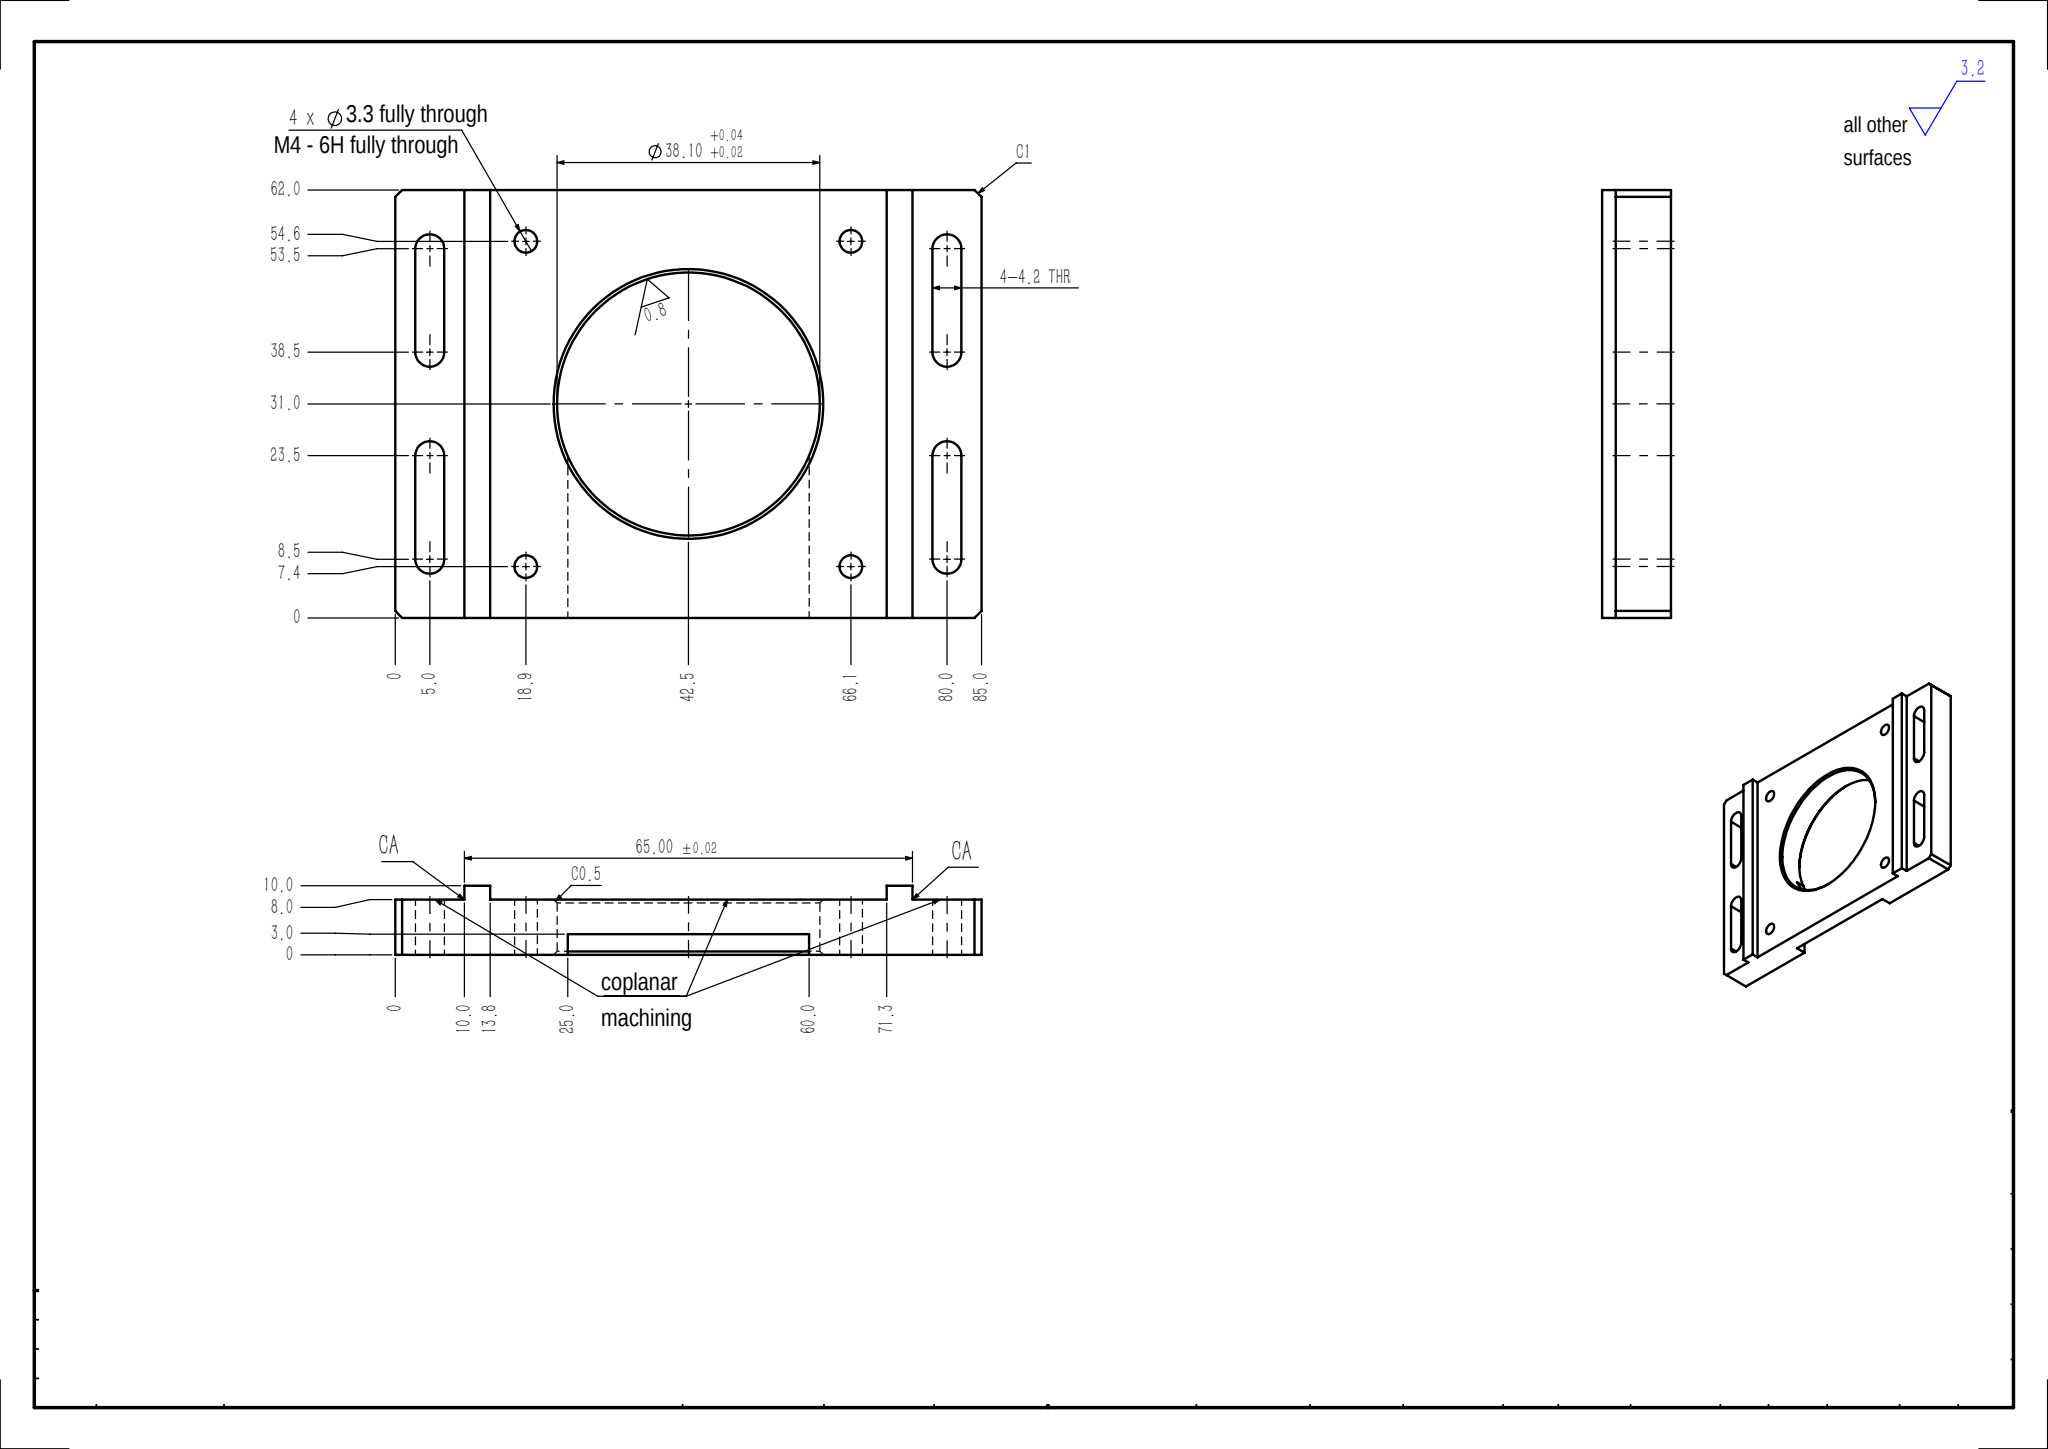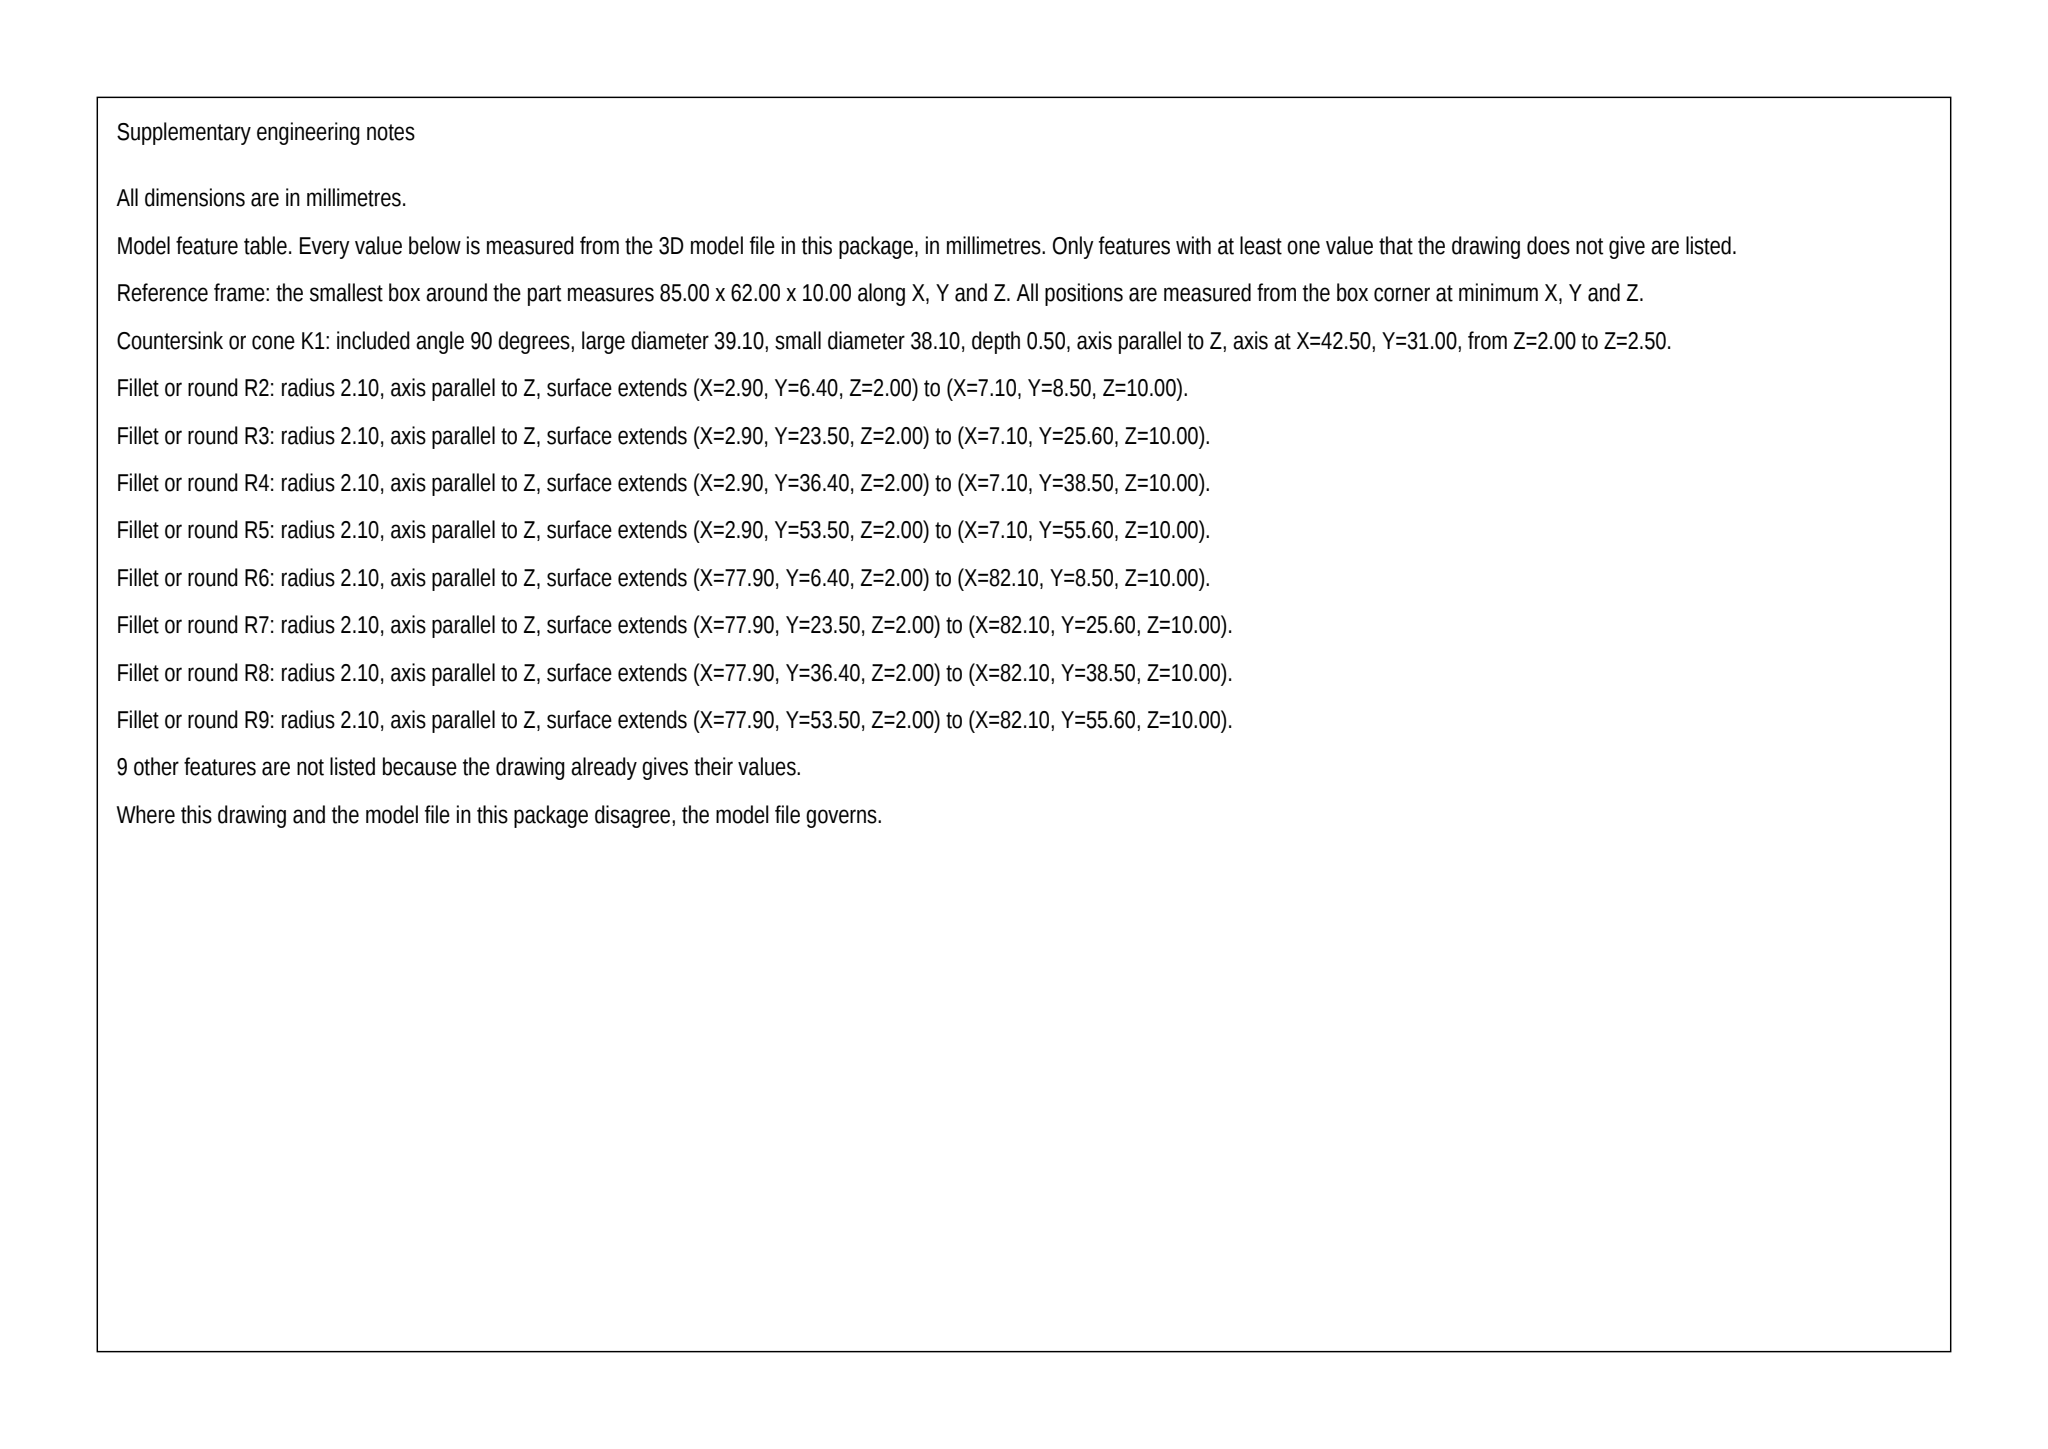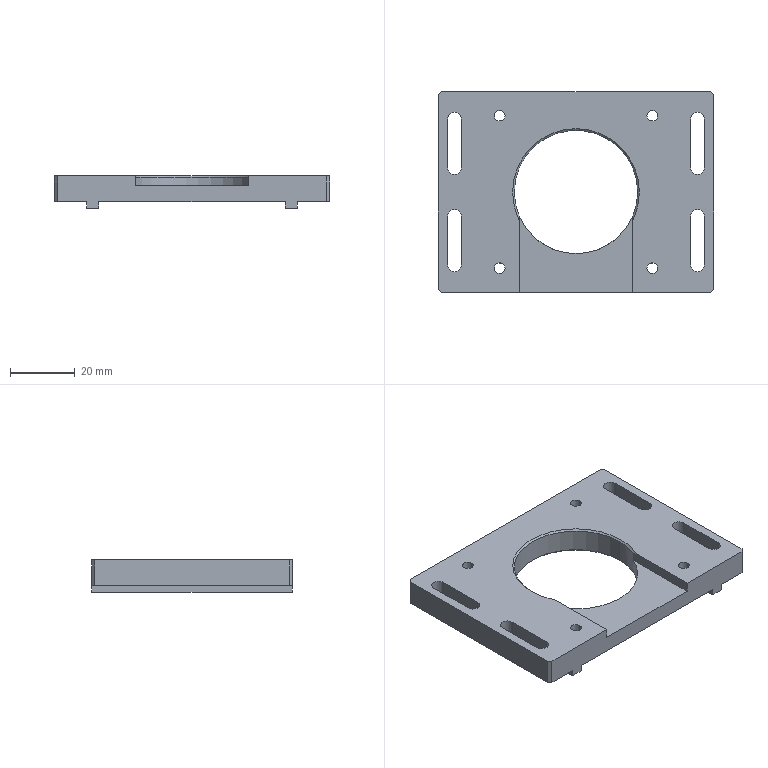Part | SolidWorks | mm | 1 solid | 52 faces | box 85 x 62 x 10 mm | volume 29604 mm3 | plane 29 | cylinder 18 | cone 5 | commonest cylinder face diameters 3.3 x8 4.2 x8 38.1 x2
build123d program:
from build123d import *

# Parameters (mm, degrees)
SKETCH1_W                  = 85
SKETCH1_H                  = 62
BOSS_EXTRUDE1_DEPTH        = 5
SKETCH2_R                  = 19.05
CUT_EXTRUDE1_DEPTH         = 54.547
M4_TAPPED_HOLE2_D          = 3.3
SKETCH12_W                 = 57.5
SKETCH12_H                 = 62
CUT_EXTRUDE2_DEPTH         = 2
SKETCH19_W                 = 15.505
SKETCH19_H                 = 62
CUT_EXTRUDE7_DEPTH         = 2
F_4_2_4_2_DIAMETER_HOLE1_D = 4.2
CUT_EXTRUDE8_DEPTH         = 54.547
SKETCH21_W                 = 35
SKETCH21_H                 = 31
CUT_EXTRUDE9_DEPTH         = 3
CHAMFER1_SIZE              = 1
CHAMFER2_SIZE              = 0.5


with BuildPart() as part:
    # Sketch1 → Boss-Extrude1 (new, symmetric)
    with BuildSketch(Plane.XY):
        Rectangle(SKETCH1_W, SKETCH1_H)
    extrude(amount=BOSS_EXTRUDE1_DEPTH, both=True)

    # Sketch2 → Cut-Extrude1 (cut, through all)
    with BuildSketch(Plane.XY.offset(5)):
        Circle(SKETCH2_R)
    extrude(amount=-CUT_EXTRUDE1_DEPTH, mode=Mode.SUBTRACT)

    # M4 Tapped Hole2 (through all)
    with Locations(Plane(origin=(0, 0, -5), x_dir=(-1, 0, 0), z_dir=(0, 0, -1))):
        with Locations((23.57, -23.57), (23.57, 23.57), (-23.57, 23.57), (-23.57, -23.57)):
            Hole(M4_TAPPED_HOLE2_D / 2)

    # Sketch12 → Cut-Extrude2 (cut)
    with BuildSketch(Plane(origin=(0, 0, -5), x_dir=(-1, 0, 0), z_dir=(0, 0, -1))):
        Rectangle(SKETCH12_W, SKETCH12_H)
    extrude(amount=-CUT_EXTRUDE2_DEPTH, mode=Mode.SUBTRACT)

    # Sketch19 → Cut-Extrude7 (cut)
    with BuildSketch(Plane.XY.offset(-5)):
        with Locations((-40.253, 0)):
            Rectangle(SKETCH19_W, SKETCH19_H)
        with Locations((40.253, 0)):
            Rectangle(SKETCH19_W, SKETCH19_H)
    extrude(amount=CUT_EXTRUDE7_DEPTH, mode=Mode.SUBTRACT)

    # 4.2 _4.2_ Diameter Hole1 (through all)
    with Locations(Plane(origin=(0, 0, -5), x_dir=(-1, 0, 0), z_dir=(0, 0, -1))):
        with Locations((-37.5, 15), (-37.5, -15), (37.5, -15), (37.5, 15)):
            Hole(F_4_2_4_2_DIAMETER_HOLE1_D / 2)

    # Sketch20 → Cut-Extrude8 (cut, through all)
    with BuildSketch(Plane.XY.offset(5)):
        with BuildLine():
            Line((-35.4, 22.5), (-35.4, 7.5))
            ThreePointArc((-35.4, 7.5), (-37.5, 5.4), (-39.6, 7.5))
            Line((-39.6, 7.5), (-39.6, 22.5))
            ThreePointArc((-39.6, 22.5), (-37.5, 24.6), (-35.4, 22.5))
        make_face()
        with BuildLine():
            Line((-35.4, -7.5), (-35.4, -22.5))
            ThreePointArc((-35.4, -22.5), (-37.5, -24.6), (-39.6, -22.5))
            Line((-39.6, -22.5), (-39.6, -7.5))
            ThreePointArc((-39.6, -7.5), (-37.5, -5.4), (-35.4, -7.5))
        make_face()
        with BuildLine():
            Line((39.6, 22.5), (39.6, 7.5))
            ThreePointArc((39.6, 7.5), (37.5, 5.4), (35.4, 7.5))
            Line((35.4, 7.5), (35.4, 22.5))
            ThreePointArc((35.4, 22.5), (37.5, 24.6), (39.6, 22.5))
        make_face()
        with BuildLine():
            Line((39.6, -7.5), (39.6, -22.5))
            ThreePointArc((39.6, -22.5), (37.5, -24.6), (35.4, -22.5))
            Line((35.4, -22.5), (35.4, -7.5))
            ThreePointArc((35.4, -7.5), (37.5, -5.4), (39.6, -7.5))
        make_face()
    extrude(amount=-CUT_EXTRUDE8_DEPTH, mode=Mode.SUBTRACT)

    # Sketch21 → Cut-Extrude9 (cut)
    with BuildSketch(Plane.XY.offset(5)):
        with Locations((0, -15.5)):
            Rectangle(SKETCH21_W, SKETCH21_H)
    extrude(amount=-CUT_EXTRUDE9_DEPTH, mode=Mode.SUBTRACT)

    # Chamfer1
    chamfer1_edges = [part.edges().sort_by_distance(p)[0] for p in [
        (42.5, -31, 1),
        (-42.5, -31, 1),
        (-42.5, 31, 1),
        (42.5, 31, 1),
    ]]
    chamfer(chamfer1_edges, length=CHAMFER1_SIZE)

    # Chamfer2
    chamfer2_edges = [part.edges().sort_by_distance(p)[0] for p in [
        (-3.842, 18.658, 5),
        (-19.05, 0, -3),
    ]]
    chamfer(chamfer2_edges, length=CHAMFER2_SIZE)


solid = part.part